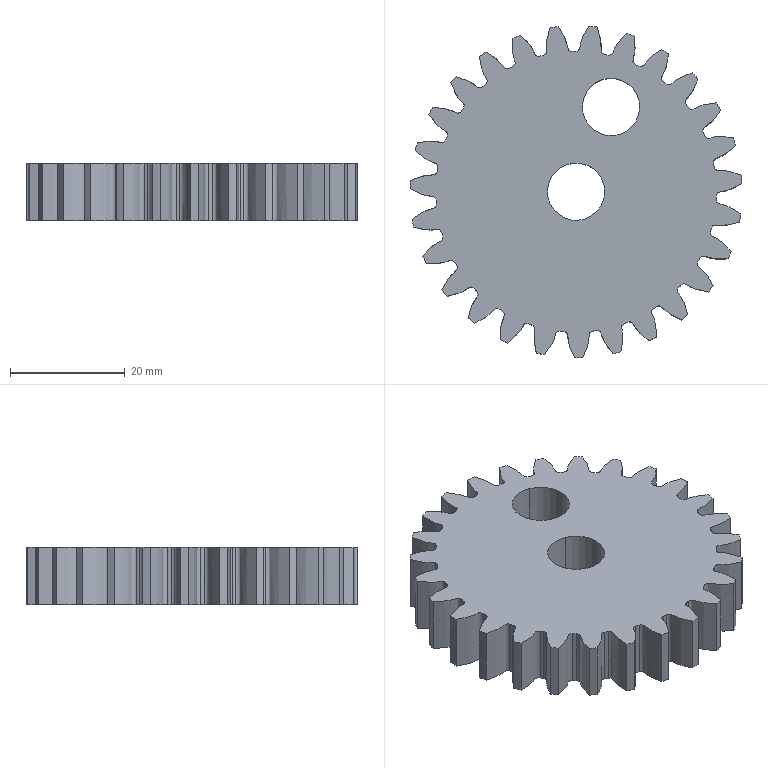Component | SolidWorks | CylindricalGear27x2Large-1 | 1 solid | 114 faces | volume 20987 mm3 | cylinder 58 | spline 54 | plane 2 | commonest cylinder face diameters 58 x27 49 x27 10 x4